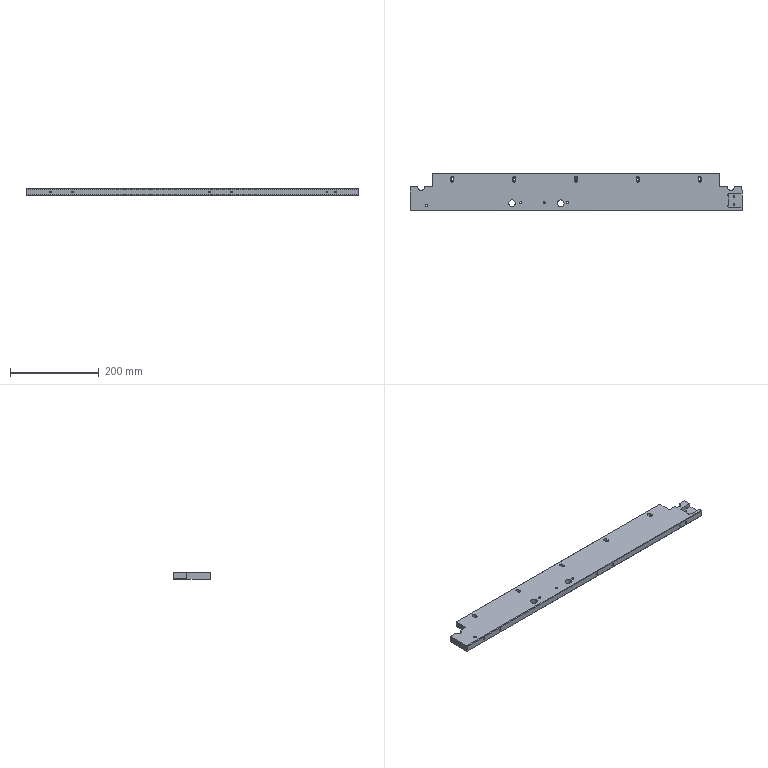Component | SolidWorks | XT-1-01-2-1 | 1 solid | 129 faces | box 750 x 85 x 15 mm | volume 884214 mm3 | cylinder 60 | plane 49 | cone 20 | commonest cylinder face diameters 4.2 x20 4.5 x10 8 x10 5 x6 15 x6 3.3 x4 6 x2 4 x2
build123d program:
from build123d import *
from OCP.BRepFilletAPI import BRepFilletAPI_MakeChamfer

# Parameters (mm, degrees)
SKETCH1_W                                       = 750
SKETCH1_H                                       = 85
BOSS_EXTRUDE1_DEPTH                             = 15
SKETCH2_R                                       = 7.5
SKETCH2_W                                       = 50
SKETCH2_H                                       = 31
CUT_EXTRUDE1_DEPTH                              = 755.95
SKETCH3_R                                       = 7.5
CUT_EXTRUDE2_DEPTH                              = 755.95
M5_TAPPED_HOLE1_D                               = 4.2
M5_TAPPED_HOLE1_DEPTH                           = 15
M5_TAPPED_HOLE1_TIP                             = 1.262
SKETCH6_W                                       = 30
SKETCH6_H                                       = 30
CUT_EXTRUDE3_DEPTH                              = 8
M6_TAPPED_HOLE1_D                               = 5
M6_TAPPED_HOLE1_DEPTH                           = 15
M6_TAPPED_HOLE1_TIP                             = 1.502
M4_HEX_SOCKET_HEAD_CAP_SCREW_CBORE1_D           = 4.5
M4_HEX_SOCKET_HEAD_CAP_SCREW_CBORE1_CBORE_D     = 8
M4_HEX_SOCKET_HEAD_CAP_SCREW_CBORE1_CBORE_DEPTH = 4.4
M5_TAPPED_HOLE2_D                               = 4.2
M5_TAPPED_HOLE2_DEPTH                           = 15
M5_TAPPED_HOLE2_TIP                             = 1.262
CUT_EXTRUDE4_DEPTH                              = 755.95
CUT_EXTRUDE5_DEPTH                              = 7
F_6_0_6_DIAMETER_HOLE1_D                        = 6
SKETCH17_R                                      = 2
CUT_EXTRUDE6_DEPTH                              = 8
CHAMFER1_SIZE                                   = 2
CHAMFER1_SIZE2                                  = 10
CHAMFER2_SIZE                                   = 1
CHAMFER3_SIZE                                   = 1
M4_TAPPED_HOLE1_D                               = 3.3
M4_TAPPED_HOLE1_DEPTH                           = 10.1
M4_TAPPED_HOLE1_TIP                             = 0.9914


with BuildPart() as part:
    # Sketch1 → Boss-Extrude1 (new body)
    with BuildSketch(Plane.XY):
        with Locations((375, -42.5)):
            Rectangle(SKETCH1_W, SKETCH1_H)
    extrude(amount=BOSS_EXTRUDE1_DEPTH)

    # Sketch2 → Cut-Extrude1 (cut, through all)
    with BuildSketch(Plane.XY.offset(15)):
        with Locations((230.5, -68)):
            Circle(SKETCH2_R)
        with Locations((340.5, -68)):
            Circle(SKETCH2_R)
        with Locations((25, -15.5)):
            Rectangle(SKETCH2_W, SKETCH2_H)
        with Locations((725, -15.5)):
            Rectangle(SKETCH2_W, SKETCH2_H)
    extrude(amount=-CUT_EXTRUDE1_DEPTH, mode=Mode.SUBTRACT)

    # Sketch3 → Cut-Extrude2 (cut, through all)
    with BuildSketch(Plane.XY.offset(15)):
        with Locations((25, -31)):
            Circle(SKETCH3_R)
        with Locations((725, -31)):
            Circle(SKETCH3_R)
    extrude(amount=-CUT_EXTRUDE2_DEPTH, mode=Mode.SUBTRACT)

    # M5 Tapped Hole1
    with Locations(Plane(origin=(0, -31, 0), x_dir=(1, 0, 0), z_dir=(0, 1, 0))):
        with Locations((9.5, -7.5), (40.5, -7.5), (709.5, -7.5), (740.5, -7.5)):
            Hole(M5_TAPPED_HOLE1_D / 2, depth=M5_TAPPED_HOLE1_DEPTH)
            with Locations((0, 0, -(M5_TAPPED_HOLE1_DEPTH + M5_TAPPED_HOLE1_TIP / 2))):  # 118° drill point
                Cone(0, M5_TAPPED_HOLE1_D / 2, M5_TAPPED_HOLE1_TIP, mode=Mode.SUBTRACT)

    # Sketch6 → Cut-Extrude3 (cut)
    with BuildSketch(Plane.XY.offset(15)):
        with Locations((735, -62)):
            Rectangle(SKETCH6_W, SKETCH6_H)
    extrude(amount=-CUT_EXTRUDE3_DEPTH, mode=Mode.SUBTRACT)

    # M6 Tapped Hole1
    with Locations(Plane.XY.offset(15)):
        with Locations((250, -67), (303, -67), (356, -67)):
            Hole(M6_TAPPED_HOLE1_D / 2, depth=M6_TAPPED_HOLE1_DEPTH)
            with Locations((0, 0, -(M6_TAPPED_HOLE1_DEPTH + M6_TAPPED_HOLE1_TIP / 2))):  # 118° drill point
                Cone(0, M6_TAPPED_HOLE1_D / 2, M6_TAPPED_HOLE1_TIP, mode=Mode.SUBTRACT)

    # M4 Hex Socket Head Cap Screw CBORE1 (through all)
    with Locations(Plane.XY.offset(15)):
        with Locations((95, -14), (235, -14), (375, -14), (515, -14), (655, -14)):
            CounterBoreHole(M4_HEX_SOCKET_HEAD_CAP_SCREW_CBORE1_D / 2, M4_HEX_SOCKET_HEAD_CAP_SCREW_CBORE1_CBORE_D / 2, M4_HEX_SOCKET_HEAD_CAP_SCREW_CBORE1_CBORE_DEPTH)

    # M5 Tapped Hole2
    with Locations(Plane(origin=(0, -85, 0), x_dir=(-1, 0, 0), z_dir=(0, -1, 0))):
        with Locations((-700, -7.5), (-680, -7.5), (-465, -7.5), (-415, -7.5), (-105, -7.5), (-55, -7.5)):
            Hole(M5_TAPPED_HOLE2_D / 2, depth=M5_TAPPED_HOLE2_DEPTH)
            with Locations((0, 0, -(M5_TAPPED_HOLE2_DEPTH + M5_TAPPED_HOLE2_TIP / 2))):  # 118° drill point
                Cone(0, M5_TAPPED_HOLE2_D / 2, M5_TAPPED_HOLE2_TIP, mode=Mode.SUBTRACT)

    # Sketch11 → Cut-Extrude4 (cut, through all)
    with BuildSketch(Plane.XY.offset(15)):
        with BuildLine():
            Line((97.25, -11.5), (97.25, -16.5))
            ThreePointArc((97.25, -16.5), (95, -18.75), (92.75, -16.5))
            Line((92.75, -16.5), (92.75, -11.5))
            ThreePointArc((92.75, -11.5), (95, -9.25), (97.25, -11.5))
        make_face()
        with BuildLine():
            Line((237.25, -11.5), (237.25, -16.5))
            ThreePointArc((237.25, -16.5), (235, -18.75), (232.75, -16.5))
            Line((232.75, -16.5), (232.75, -11.5))
            ThreePointArc((232.75, -11.5), (235, -9.25), (237.25, -11.5))
        make_face()
        with BuildLine():
            Line((377.25, -11.5), (377.25, -16.5))
            ThreePointArc((377.25, -16.5), (375, -18.75), (372.75, -16.5))
            Line((372.75, -16.5), (372.75, -11.5))
            ThreePointArc((372.75, -11.5), (375, -9.25), (377.25, -11.5))
        make_face()
        with BuildLine():
            Line((517.25, -11.5), (517.25, -16.5))
            ThreePointArc((517.25, -16.5), (515, -18.75), (512.75, -16.5))
            Line((512.75, -16.5), (512.75, -11.5))
            ThreePointArc((512.75, -11.5), (515, -9.25), (517.25, -11.5))
        make_face()
        with BuildLine():
            Line((657.25, -11.5), (657.25, -16.5))
            ThreePointArc((657.25, -16.5), (655, -18.75), (652.75, -16.5))
            Line((652.75, -16.5), (652.75, -11.5))
            ThreePointArc((652.75, -11.5), (655, -9.25), (657.25, -11.5))
        make_face()
    extrude(amount=-CUT_EXTRUDE4_DEPTH, mode=Mode.SUBTRACT)

    # Sketch12 → Cut-Extrude5 (cut)
    with BuildSketch(Plane.XY.offset(15)):
        with BuildLine():
            Line((99, -11.5), (99, -16.5))
            ThreePointArc((99, -16.5), (95, -20.5), (91, -16.5))
            Line((91, -16.5), (91, -11.5))
            ThreePointArc((91, -11.5), (95, -7.5), (99, -11.5))
        make_face()
        with BuildLine():
            Line((239, -11.5), (239, -16.5))
            ThreePointArc((239, -16.5), (235, -20.5), (231, -16.5))
            Line((231, -16.5), (231, -11.5))
            ThreePointArc((231, -11.5), (235, -7.5), (239, -11.5))
        make_face()
        with BuildLine():
            Line((379, -11.5), (379, -16.5))
            ThreePointArc((379, -16.5), (375, -20.5), (371, -16.5))
            Line((371, -16.5), (371, -11.5))
            ThreePointArc((371, -11.5), (375, -7.5), (379, -11.5))
        make_face()
        with BuildLine():
            Line((519, -11.5), (519, -16.5))
            ThreePointArc((519, -16.5), (515, -20.5), (511, -16.5))
            Line((511, -16.5), (511, -11.5))
            ThreePointArc((511, -11.5), (515, -7.5), (519, -11.5))
        make_face()
        with BuildLine():
            Line((659, -11.5), (659, -16.5))
            ThreePointArc((659, -16.5), (655, -20.5), (651, -16.5))
            Line((651, -16.5), (651, -11.5))
            ThreePointArc((651, -11.5), (655, -7.5), (659, -11.5))
        make_face()
    extrude(amount=-CUT_EXTRUDE5_DEPTH, mode=Mode.SUBTRACT)

    # 6.0 _6_ Diameter Hole1 (through all)
    with Locations(Plane.XY.offset(15)):
        with Locations((37, -73)):
            Hole(F_6_0_6_DIAMETER_HOLE1_D / 2)

    # Sketch17 → Cut-Extrude6 (cut)
    with BuildSketch(Plane.XY.offset(15)):
        with Locations((720, -49)):
            Circle(SKETCH17_R)
        with Locations((720, -75)):
            Circle(SKETCH17_R)
    extrude(amount=-CUT_EXTRUDE6_DEPTH, mode=Mode.SUBTRACT)

    # Chamfer1: one chamfer whose edges measure the first distance from different faces: ONE call of the kernel's chamfer builder (chamfer() names one face for all edges)
    chamfer1_edges_1 = [part.edges().sort_by_distance(p)[0] for p in [
        (50, -15.5, 0),
    ]]
    chamfer1_side_1 = [part.faces().sort_by_distance(p)[0] for p in [
        (50, -15.5, 7.5),
    ]]
    chamfer1_edges_2 = [part.edges().sort_by_distance(p)[0] for p in [
        (700, -15.5, 0),
    ]]
    chamfer1_side_2 = [part.faces().sort_by_distance(p)[0] for p in [
        (700, -15.5, 7.5),
    ]]
    chamfer1 = BRepFilletAPI_MakeChamfer(part.part.solid().wrapped)
    for e in chamfer1_edges_1:
        chamfer1.Add(CHAMFER1_SIZE, CHAMFER1_SIZE2, e.wrapped, chamfer1_side_1[0].wrapped)  # the first distance lies on this face
    for e in chamfer1_edges_2:
        chamfer1.Add(CHAMFER1_SIZE, CHAMFER1_SIZE2, e.wrapped, chamfer1_side_2[0].wrapped)  # the first distance lies on this face
    add(Compound.cast(chamfer1.Shape()), mode=Mode.REPLACE)

    # Chamfer2
    chamfer2_edges = [part.edges().sort_by_distance(p)[0] for p in [
        (375, 0, 15),
        (375, 0, 0),
        (375, -85, 0),
        (375, -85, 15),
    ]]
    chamfer(chamfer2_edges, length=CHAMFER2_SIZE)

    # Chamfer3
    chamfer3_edges = [part.edges().sort_by_distance(p)[0] for p in [
        (700, 0, 8),
        (50, 0, 8),
    ]]
    chamfer(chamfer3_edges, length=CHAMFER3_SIZE)

    # M4 Tapped Hole1
    with Locations(Plane.XY.offset(7)):
        with Locations((732, -53), (732, -71)):
            Hole(M4_TAPPED_HOLE1_D / 2, depth=M4_TAPPED_HOLE1_DEPTH)
            with Locations((0, 0, -(M4_TAPPED_HOLE1_DEPTH + M4_TAPPED_HOLE1_TIP / 2))):  # 118° drill point
                Cone(0, M4_TAPPED_HOLE1_D / 2, M4_TAPPED_HOLE1_TIP, mode=Mode.SUBTRACT)


solid = part.part

# Placed as in the assembly
solid = solid.moved(Location((214.283, 139.385, -7.5), (0, 0, 0)))